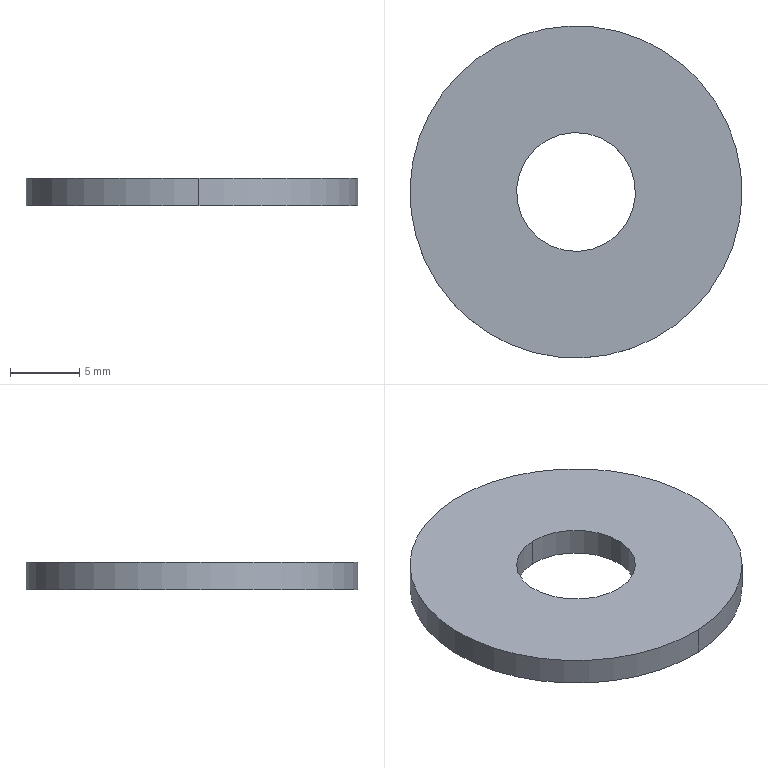Component | SolidWorks | DriveDevice-1_FlatWasher-1 | 1 solid | 6 faces | box 24 x 24 x 2 mm | volume 789 mm3 | cylinder 4 | plane 2 | commonest cylinder face diameters 8.6 x2 24 x2
build123d program:
from build123d import *

# Parameters (mm, degrees)
SKETCH1_R           = 12
SKETCH1_R_2         = 4.3
BOSS_EXTRUDE1_DEPTH = 2


with BuildPart() as part:
    # Sketch1 → Boss-Extrude1 (new body)
    with BuildSketch(Plane(origin=(0, 0, 0), x_dir=(1, 0, 0), z_dir=(0, 1, 0))):
        with Locations(Location((0, -3.983, 0), (0, 0, 270))):
            Circle(SKETCH1_R)
        with Locations(Location((0, -3.983, 0), (0, 0, 270))):
            Circle(SKETCH1_R_2, mode=Mode.SUBTRACT)
    extrude(amount=BOSS_EXTRUDE1_DEPTH)


solid = part.part

# Placed as in the assembly
solid = solid.moved(Location((55, 46.983, 53.5), (90, 0, 0)))
STEP:
#1=CARTESIAN_POINT('',(2.172,1.524,2.106));
#2=VERTEX_POINT('',#1);
#3=CARTESIAN_POINT('',(2.158,1.862,2.106));
#4=VERTEX_POINT('',#3);
#5=CARTESIAN_POINT('',(2.165,1.693,2.106));
#6=DIRECTION('',(0.,0.,-1.));
#7=DIRECTION('',(-0.04206,0.9991,0.));
#8=AXIS2_PLACEMENT_3D('',#5,#6,#7);
#9=CIRCLE('',#8,0.1693);
#10=EDGE_CURVE('',#2,#4,#9,.T.);
#11=ORIENTED_EDGE('',*,*,#10,.T.);
#12=CARTESIAN_POINT('',(2.158,1.862,2.185));
#13=VERTEX_POINT('',#12);
#14=CARTESIAN_POINT('',(2.158,1.862,2.106));
#15=DIRECTION('',(0.,0.,1.));
#16=VECTOR('',#15,39.37);
#17=LINE('',#14,#16);
#18=EDGE_CURVE('',#4,#13,#17,.T.);
#19=ORIENTED_EDGE('',*,*,#18,.T.);
#20=CARTESIAN_POINT('',(2.172,1.524,2.185));
#21=VERTEX_POINT('',#20);
#22=CARTESIAN_POINT('',(2.165,1.693,2.185));
#23=DIRECTION('',(0.,0.,-1.));
#24=DIRECTION('',(-0.04206,0.9991,0.));
#25=AXIS2_PLACEMENT_3D('',#22,#23,#24);
#26=CIRCLE('',#25,0.1693);
#27=EDGE_CURVE('',#21,#13,#26,.T.);
#28=ORIENTED_EDGE('',*,*,#27,.F.);
#29=CARTESIAN_POINT('',(2.172,1.524,2.106));
#30=DIRECTION('',(0.,0.,1.));
#31=VECTOR('',#30,39.37);
#32=LINE('',#29,#31);
#33=EDGE_CURVE('',#2,#21,#32,.T.);
#34=ORIENTED_EDGE('',*,*,#33,.F.);
#35=EDGE_LOOP('',(#11,#19,#28,#34));
#36=FACE_OUTER_BOUND('',#35,.T.);
#37=CARTESIAN_POINT('',(2.165,1.693,2.106));
#38=DIRECTION('',(0.,0.,1.));
#39=DIRECTION('',(0.04206,-0.9991,0.));
#40=AXIS2_PLACEMENT_3D('',#37,#38,#39);
#41=CYLINDRICAL_SURFACE('',#40,0.1693);
#42=ADVANCED_FACE('',(#36),#41,.F.);
#43=CARTESIAN_POINT('',(2.145,2.165,2.106));
#44=VERTEX_POINT('',#43);
#45=CARTESIAN_POINT('',(2.185,1.221,2.106));
#46=VERTEX_POINT('',#45);
#47=CARTESIAN_POINT('',(2.165,1.693,2.106));
#48=DIRECTION('',(0.,0.,-1.));
#49=DIRECTION('',(-0.04206,0.9991,0.));
#50=AXIS2_PLACEMENT_3D('',#47,#48,#49);
#51=CIRCLE('',#50,0.4724);
#52=EDGE_CURVE('',#44,#46,#51,.T.);
#53=ORIENTED_EDGE('',*,*,#52,.F.);
#54=CARTESIAN_POINT('',(2.145,2.165,2.185));
#55=VERTEX_POINT('',#54);
#56=CARTESIAN_POINT('',(2.145,2.165,2.106));
#57=DIRECTION('',(0.,0.,1.));
#58=VECTOR('',#57,39.37);
#59=LINE('',#56,#58);
#60=EDGE_CURVE('',#44,#55,#59,.T.);
#61=ORIENTED_EDGE('',*,*,#60,.T.);
#62=CARTESIAN_POINT('',(2.185,1.221,2.185));
#63=VERTEX_POINT('',#62);
#64=CARTESIAN_POINT('',(2.165,1.693,2.185));
#65=DIRECTION('',(0.,0.,-1.));
#66=DIRECTION('',(-0.04206,0.9991,0.));
#67=AXIS2_PLACEMENT_3D('',#64,#65,#66);
#68=CIRCLE('',#67,0.4724);
#69=EDGE_CURVE('',#55,#63,#68,.T.);
#70=ORIENTED_EDGE('',*,*,#69,.T.);
#71=CARTESIAN_POINT('',(2.185,1.221,2.106));
#72=DIRECTION('',(0.,0.,1.));
#73=VECTOR('',#72,39.37);
#74=LINE('',#71,#73);
#75=EDGE_CURVE('',#46,#63,#74,.T.);
#76=ORIENTED_EDGE('',*,*,#75,.F.);
#77=EDGE_LOOP('',(#53,#61,#70,#76));
#78=FACE_OUTER_BOUND('',#77,.T.);
#79=CARTESIAN_POINT('',(2.165,1.693,2.106));
#80=DIRECTION('',(0.,0.,1.));
#81=DIRECTION('',(0.04206,-0.9991,0.));
#82=AXIS2_PLACEMENT_3D('',#79,#80,#81);
#83=CYLINDRICAL_SURFACE('',#82,0.4724);
#84=ADVANCED_FACE('',(#78),#83,.T.);
#85=CARTESIAN_POINT('',(2.165,1.693,2.106));
#86=DIRECTION('',(0.,0.,-1.));
#87=DIRECTION('',(-0.04206,0.9991,0.));
#88=AXIS2_PLACEMENT_3D('',#85,#86,#87);
#89=CIRCLE('',#88,0.4724);
#90=EDGE_CURVE('',#46,#44,#89,.T.);
#91=ORIENTED_EDGE('',*,*,#90,.T.);
#92=ORIENTED_EDGE('',*,*,#52,.T.);
#93=EDGE_LOOP('',(#91,#92));
#94=FACE_OUTER_BOUND('',#93,.T.);
#95=ORIENTED_EDGE('',*,*,#10,.F.);
#96=CARTESIAN_POINT('',(2.165,1.693,2.106));
#97=DIRECTION('',(0.,0.,-1.));
#98=DIRECTION('',(-0.04206,0.9991,0.));
#99=AXIS2_PLACEMENT_3D('',#96,#97,#98);
#100=CIRCLE('',#99,0.1693);
#101=EDGE_CURVE('',#4,#2,#100,.T.);
#102=ORIENTED_EDGE('',*,*,#101,.F.);
#103=EDGE_LOOP('',(#95,#102));
#104=FACE_BOUND('',#103,.T.);
#105=CARTESIAN_POINT('',(2.165,1.693,2.106));
#106=DIRECTION('',(0.,0.,-1.));
#107=DIRECTION('',(-0.04206,0.9991,0.));
#108=AXIS2_PLACEMENT_3D('',#105,#106,#107);
#109=PLANE('',#108);
#110=ADVANCED_FACE('',(#94,#104),#109,.T.);
#111=CARTESIAN_POINT('',(2.165,1.693,2.185));
#112=DIRECTION('',(0.,0.,-1.));
#113=DIRECTION('',(-0.04206,0.9991,0.));
#114=AXIS2_PLACEMENT_3D('',#111,#112,#113);
#115=CIRCLE('',#114,0.4724);
#116=EDGE_CURVE('',#63,#55,#115,.T.);
#117=ORIENTED_EDGE('',*,*,#116,.F.);
#118=ORIENTED_EDGE('',*,*,#69,.F.);
#119=EDGE_LOOP('',(#117,#118));
#120=FACE_OUTER_BOUND('',#119,.T.);
#121=ORIENTED_EDGE('',*,*,#27,.T.);
#122=CARTESIAN_POINT('',(2.165,1.693,2.185));
#123=DIRECTION('',(0.,0.,-1.));
#124=DIRECTION('',(-0.04206,0.9991,0.));
#125=AXIS2_PLACEMENT_3D('',#122,#123,#124);
#126=CIRCLE('',#125,0.1693);
#127=EDGE_CURVE('',#13,#21,#126,.T.);
#128=ORIENTED_EDGE('',*,*,#127,.T.);
#129=EDGE_LOOP('',(#121,#128));
#130=FACE_BOUND('',#129,.T.);
#131=CARTESIAN_POINT('',(2.165,1.693,2.185));
#132=DIRECTION('',(0.,0.,-1.));
#133=DIRECTION('',(-0.04206,0.9991,0.));
#134=AXIS2_PLACEMENT_3D('',#131,#132,#133);
#135=PLANE('',#134);
#136=ADVANCED_FACE('',(#120,#130),#135,.F.);
#137=ORIENTED_EDGE('',*,*,#60,.F.);
#138=ORIENTED_EDGE('',*,*,#90,.F.);
#139=ORIENTED_EDGE('',*,*,#75,.T.);
#140=ORIENTED_EDGE('',*,*,#116,.T.);
#141=EDGE_LOOP('',(#137,#138,#139,#140));
#142=FACE_OUTER_BOUND('',#141,.T.);
#143=CARTESIAN_POINT('',(2.165,1.693,2.106));
#144=DIRECTION('',(0.,0.,1.));
#145=DIRECTION('',(0.04206,-0.9991,0.));
#146=AXIS2_PLACEMENT_3D('',#143,#144,#145);
#147=CYLINDRICAL_SURFACE('',#146,0.4724);
#148=ADVANCED_FACE('',(#142),#147,.T.);
#149=ORIENTED_EDGE('',*,*,#18,.F.);
#150=ORIENTED_EDGE('',*,*,#101,.T.);
#151=ORIENTED_EDGE('',*,*,#33,.T.);
#152=ORIENTED_EDGE('',*,*,#127,.F.);
#153=EDGE_LOOP('',(#149,#150,#151,#152));
#154=FACE_OUTER_BOUND('',#153,.T.);
#155=CARTESIAN_POINT('',(2.165,1.693,2.106));
#156=DIRECTION('',(0.,0.,1.));
#157=DIRECTION('',(0.04206,-0.9991,0.));
#158=AXIS2_PLACEMENT_3D('',#155,#156,#157);
#159=CYLINDRICAL_SURFACE('',#158,0.1693);
#160=ADVANCED_FACE('',(#154),#159,.F.);
#161=CLOSED_SHELL('',(#42,#84,#110,#136,#148,#160));
#162=MANIFOLD_SOLID_BREP('',#161);
#163=CARTESIAN_POINT('',(0.,0.,0.));
#164=DIRECTION('',(0.,0.,1.));
#165=DIRECTION('',(1.,0.,0.));
#166=AXIS2_PLACEMENT_3D('',#163,#164,#165);
#167=(LENGTH_UNIT()NAMED_UNIT(*)SI_UNIT($,.METRE.));
#168=LENGTH_MEASURE_WITH_UNIT(LENGTH_MEASURE(0.0254),#167);
#169=DIMENSIONAL_EXPONENTS(1.,0.,0.,0.,0.,0.,0.);
#170=(CONVERSION_BASED_UNIT('',#168)LENGTH_UNIT()NAMED_UNIT(#169));
#171=UNCERTAINTY_MEASURE_WITH_UNIT(LENGTH_MEASURE(0.00001),#170,'','');
#172=(NAMED_UNIT(*)PLANE_ANGLE_UNIT()SI_UNIT($,.RADIAN.));
#173=(NAMED_UNIT(*)SI_UNIT($,.STERADIAN.)SOLID_ANGLE_UNIT());
#174=(GEOMETRIC_REPRESENTATION_CONTEXT(3)GLOBAL_UNCERTAINTY_ASSIGNED_CONTEXT((#171))GLOBAL_UNIT_ASSIGNED_CONTEXT((#170,#172,#173))REPRESENTATION_CONTEXT('',''));
#175=ADVANCED_BREP_SHAPE_REPRESENTATION('',(#162,#166),#174);
#176=COLOUR_RGB('',0.7922,0.8196,0.9333);
#177=FILL_AREA_STYLE_COLOUR('',#176);
#178=FILL_AREA_STYLE('',(#177));
#179=SURFACE_STYLE_FILL_AREA(#178);
#180=SURFACE_SIDE_STYLE('',(#179));
#181=SURFACE_STYLE_USAGE(.BOTH.,#180);
#182=PRESENTATION_STYLE_ASSIGNMENT((#181));
#183=STYLED_ITEM('',(#182),#162);
#184=PRESENTATION_LAYER_ASSIGNMENT('','',(#183));
#185=(LENGTH_UNIT()NAMED_UNIT(*)SI_UNIT($,.METRE.));
#186=LENGTH_MEASURE_WITH_UNIT(LENGTH_MEASURE(0.0254),#185);
#187=DIMENSIONAL_EXPONENTS(1.,0.,0.,0.,0.,0.,0.);
#188=(CONVERSION_BASED_UNIT('',#186)LENGTH_UNIT()NAMED_UNIT(#187));
#189=UNCERTAINTY_MEASURE_WITH_UNIT(LENGTH_MEASURE(0.00001),#188,'','');
#190=(NAMED_UNIT(*)PLANE_ANGLE_UNIT()SI_UNIT($,.RADIAN.));
#191=(NAMED_UNIT(*)SI_UNIT($,.STERADIAN.)SOLID_ANGLE_UNIT());
#192=(GEOMETRIC_REPRESENTATION_CONTEXT(3)GLOBAL_UNCERTAINTY_ASSIGNED_CONTEXT((#189))GLOBAL_UNIT_ASSIGNED_CONTEXT((#188,#190,#191))REPRESENTATION_CONTEXT('',''));
#193=MECHANICAL_DESIGN_GEOMETRIC_PRESENTATION_REPRESENTATION('',(#183),#192);